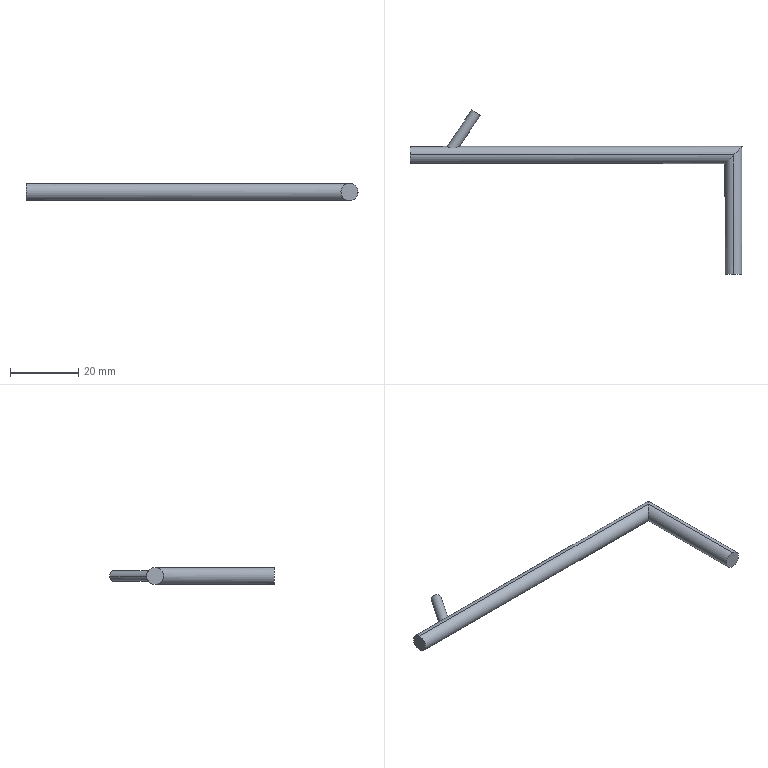Component | SolidWorks | PistonRod-1 | 1 solid | 9 faces | box 97.5 x 48.27 x 5 mm | volume 2638 mm3 | cylinder 6 | plane 3 | commonest cylinder face diameters 5 x4 3 x2
build123d program:
from build123d import *

# Parameters (mm, degrees)
SWEEP1_PROFILE_R = 2.5
SWEEP2_PROFILE_R = 1.5


with BuildPart() as part:
    # Sweep1: sweep along a path in Sketch1
    with BuildLine(Plane.XY) as sweep1_path:
        Line((35, 0), (0, 0))
        Line((0, 0), (0, 95))
    # Sweep1 profile (on start of the path) → Sweep1 (sweep)
    with BuildSketch(Plane(origin=(35, 0, 0), x_dir=(0, 0, -1), z_dir=(-1, 0, 0))):
        Circle(SWEEP1_PROFILE_R)
    sweep(path=sweep1_path.line, transition=Transition.RIGHT)

    # Sweep2: sweep along a path in Sketch2
    with BuildLine(Plane.XY) as sweep2_path:
        Line((0, 84), (-12.436, 75.612))
    # Sweep2 profile (on start of the path) → Sweep2 (sweep)
    with BuildSketch(Plane(origin=(0, 84, 0), x_dir=(0.5592, -0.829, 0), z_dir=(-0.829, -0.5592, 0))):
        Circle(SWEEP2_PROFILE_R)
    sweep(path=sweep2_path.line)


solid = part.part

# Placed as in the assembly
solid = solid.moved(Location((-25, -95, 0), (180, 0, 90)))
STEP:
#1=COLOUR_RGB('',0.7922,0.8196,0.9333);
#2=FILL_AREA_STYLE_COLOUR('',#1);
#3=FILL_AREA_STYLE('',(#2));
#4=SURFACE_STYLE_FILL_AREA(#3);
#5=SURFACE_SIDE_STYLE('',(#4));
#6=SURFACE_STYLE_USAGE(.BOTH.,#5);
#7=PRESENTATION_STYLE_ASSIGNMENT((#6));
#8=CARTESIAN_POINT('',(-4.296,-3.642,0.));
#9=VERTEX_POINT('',#8);
#10=CARTESIAN_POINT('',(-4.154,-3.642,0.));
#11=VERTEX_POINT('',#10);
#12=CARTESIAN_POINT('',(-4.296,-3.642,0.));
#13=CARTESIAN_POINT('',(-4.296,-3.642,-0.00441));
#14=CARTESIAN_POINT('',(-4.296,-3.642,-0.008751));
#15=CARTESIAN_POINT('',(-4.294,-3.643,-0.0173));
#16=CARTESIAN_POINT('',(-4.293,-3.644,-0.02152));
#17=CARTESIAN_POINT('',(-4.288,-3.647,-0.03335));
#18=CARTESIAN_POINT('',(-4.284,-3.65,-0.04043));
#19=CARTESIAN_POINT('',(-4.274,-3.655,-0.04863));
#20=CARTESIAN_POINT('',(-4.271,-3.656,-0.05101));
#21=CARTESIAN_POINT('',(-4.263,-3.658,-0.05476));
#22=CARTESIAN_POINT('',(-4.259,-3.659,-0.05621));
#23=CARTESIAN_POINT('',(-4.247,-3.661,-0.05921));
#24=CARTESIAN_POINT('',(-4.238,-3.662,-0.05945));
#25=CARTESIAN_POINT('',(-4.22,-3.66,-0.05769));
#26=CARTESIAN_POINT('',(-4.212,-3.659,-0.05569));
#27=CARTESIAN_POINT('',(-4.196,-3.655,-0.05005));
#28=CARTESIAN_POINT('',(-4.188,-3.653,-0.04641));
#29=CARTESIAN_POINT('',(-4.177,-3.65,-0.03937));
#30=CARTESIAN_POINT('',(-4.174,-3.649,-0.03679));
#31=CARTESIAN_POINT('',(-4.168,-3.647,-0.03105));
#32=CARTESIAN_POINT('',(-4.165,-3.646,-0.02785));
#33=CARTESIAN_POINT('',(-4.157,-3.643,-0.01739));
#34=CARTESIAN_POINT('',(-4.154,-3.642,-0.008908));
#35=CARTESIAN_POINT('',(-4.154,-3.642,0.));
#36=B_SPLINE_CURVE_WITH_KNOTS('',3,(#12,#13,#14,#15,#16,#17,#18,#19,#20,#21,#22,#23,#24,#25,#26,#27,#28,#29,#30,#31,#32,#33,#34,#35),.UNSPECIFIED.,.F.,.F.,(4,2,2,2,2,2,2,2,2,2,2,4),(0.005318,0.00565,0.005983,0.006647,0.00698,0.007312,0.007977,0.008641,0.009306,0.009638,0.00997,0.01064),.UNSPECIFIED.);
#37=EDGE_CURVE('',#9,#11,#36,.T.);
#38=ORIENTED_EDGE('',*,*,#37,.F.);
#39=CARTESIAN_POINT('',(-4.01,-3.218,0.));
#40=VERTEX_POINT('',#39);
#41=CARTESIAN_POINT('',(-4.34,-3.707,0.));
#42=DIRECTION('',(0.5592,0.829,-0.));
#43=VECTOR('',#42,39.37);
#44=LINE('',#41,#43);
#45=EDGE_CURVE('',#9,#40,#44,.T.);
#46=ORIENTED_EDGE('',*,*,#45,.T.);
#47=CARTESIAN_POINT('',(-3.912,-3.284,0.));
#48=VERTEX_POINT('',#47);
#49=CARTESIAN_POINT('',(-3.961,-3.251,0.));
#50=DIRECTION('',(0.5592,0.829,-0.));
#51=DIRECTION('',(0.829,-0.5592,-0.));
#52=AXIS2_PLACEMENT_3D('',#49,#50,#51);
#53=CIRCLE('',#52,0.05906);
#54=EDGE_CURVE('',#48,#40,#53,.T.);
#55=ORIENTED_EDGE('',*,*,#54,.F.);
#56=CARTESIAN_POINT('',(-4.242,-3.773,0.));
#57=DIRECTION('',(0.5592,0.829,-0.));
#58=VECTOR('',#57,39.37);
#59=LINE('',#56,#58);
#60=EDGE_CURVE('',#11,#48,#59,.T.);
#61=ORIENTED_EDGE('',*,*,#60,.F.);
#62=EDGE_LOOP('',(#38,#46,#55,#61));
#63=FACE_OUTER_BOUND('',#62,.T.);
#64=CARTESIAN_POINT('',(-4.291,-3.74,0.));
#65=DIRECTION('',(0.5592,0.829,-0.));
#66=DIRECTION('',(0.829,-0.5592,-0.));
#67=AXIS2_PLACEMENT_3D('',#64,#65,#66);
#68=CYLINDRICAL_SURFACE('',#67,0.05906);
#69=ADVANCED_FACE('',(#63),#68,.T.);
#70=CARTESIAN_POINT('',(-0.9843,-5.118,0.09843));
#71=VERTEX_POINT('',#70);
#72=CARTESIAN_POINT('',(-0.9843,-5.118,-0.09843));
#73=VERTEX_POINT('',#72);
#74=CARTESIAN_POINT('',(-0.9843,-5.118,0.));
#75=DIRECTION('',(0.,-1.,0.));
#76=DIRECTION('',(0.,0.,1.));
#77=AXIS2_PLACEMENT_3D('',#74,#75,#76);
#78=CIRCLE('',#77,0.09843);
#79=EDGE_CURVE('',#71,#73,#78,.T.);
#80=ORIENTED_EDGE('',*,*,#79,.F.);
#81=CARTESIAN_POINT('',(-0.9843,-3.74,0.09843));
#82=VERTEX_POINT('',#81);
#83=CARTESIAN_POINT('',(-0.9843,-5.118,0.09843));
#84=DIRECTION('',(0.,1.,-0.));
#85=VECTOR('',#84,39.37);
#86=LINE('',#83,#85);
#87=EDGE_CURVE('',#71,#82,#86,.T.);
#88=ORIENTED_EDGE('',*,*,#87,.T.);
#89=CARTESIAN_POINT('',(-0.9843,-3.74,-0.09843));
#90=VERTEX_POINT('',#89);
#91=CARTESIAN_POINT('',(-0.9843,-3.74,-0.09843));
#92=CARTESIAN_POINT('',(-1.181,-3.937,-0.09843));
#93=CARTESIAN_POINT('',(-1.181,-3.937,0.09843));
#94=CARTESIAN_POINT('',(-0.9843,-3.74,0.09843));
#95=(BOUNDED_CURVE()B_SPLINE_CURVE(3,(#91,#92,#93,#94),.UNSPECIFIED.,.F.,.T.)B_SPLINE_CURVE_WITH_KNOTS((4,4),(1.571,4.712),.UNSPECIFIED.)CURVE()GEOMETRIC_REPRESENTATION_ITEM()RATIONAL_B_SPLINE_CURVE((1.,0.3333,0.3333,1.))REPRESENTATION_ITEM(''));
#96=EDGE_CURVE('',#90,#82,#95,.T.);
#97=ORIENTED_EDGE('',*,*,#96,.F.);
#98=CARTESIAN_POINT('',(-0.9843,-5.118,-0.09843));
#99=DIRECTION('',(0.,1.,-0.));
#100=VECTOR('',#99,39.37);
#101=LINE('',#98,#100);
#102=EDGE_CURVE('',#73,#90,#101,.T.);
#103=ORIENTED_EDGE('',*,*,#102,.F.);
#104=EDGE_LOOP('',(#80,#88,#97,#103));
#105=FACE_OUTER_BOUND('',#104,.T.);
#106=CARTESIAN_POINT('',(-0.9843,-5.118,0.));
#107=DIRECTION('',(0.,1.,-0.));
#108=DIRECTION('',(0.,0.,-1.));
#109=AXIS2_PLACEMENT_3D('',#106,#107,#108);
#110=CYLINDRICAL_SURFACE('',#109,0.09843);
#111=ADVANCED_FACE('',(#105),#110,.T.);
#112=ORIENTED_EDGE('',*,*,#96,.T.);
#113=CARTESIAN_POINT('',(-4.724,-3.74,0.09843));
#114=VERTEX_POINT('',#113);
#115=CARTESIAN_POINT('',(-0.7638,-3.74,0.09843));
#116=DIRECTION('',(-1.,-0.,0.));
#117=VECTOR('',#116,39.37);
#118=LINE('',#115,#117);
#119=EDGE_CURVE('',#82,#114,#118,.T.);
#120=ORIENTED_EDGE('',*,*,#119,.T.);
#121=CARTESIAN_POINT('',(-4.724,-3.74,-0.09843));
#122=VERTEX_POINT('',#121);
#123=CARTESIAN_POINT('',(-4.724,-3.74,0.));
#124=DIRECTION('',(1.,0.,-0.));
#125=DIRECTION('',(0.,0.,1.));
#126=AXIS2_PLACEMENT_3D('',#123,#124,#125);
#127=CIRCLE('',#126,0.09843);
#128=EDGE_CURVE('',#114,#122,#127,.T.);
#129=ORIENTED_EDGE('',*,*,#128,.T.);
#130=CARTESIAN_POINT('',(-0.7638,-3.74,-0.09843));
#131=DIRECTION('',(-1.,-0.,0.));
#132=VECTOR('',#131,39.37);
#133=LINE('',#130,#132);
#134=EDGE_CURVE('',#90,#122,#133,.T.);
#135=ORIENTED_EDGE('',*,*,#134,.F.);
#136=EDGE_LOOP('',(#112,#120,#129,#135));
#137=FACE_OUTER_BOUND('',#136,.T.);
#138=CARTESIAN_POINT('',(-0.7638,-3.74,0.));
#139=DIRECTION('',(-1.,-0.,0.));
#140=DIRECTION('',(0.,0.,-1.));
#141=AXIS2_PLACEMENT_3D('',#138,#139,#140);
#142=CYLINDRICAL_SURFACE('',#141,0.09843);
#143=ADVANCED_FACE('',(#137),#142,.T.);
#144=ORIENTED_EDGE('',*,*,#87,.F.);
#145=CARTESIAN_POINT('',(-0.9843,-5.118,0.));
#146=DIRECTION('',(0.,-1.,0.));
#147=DIRECTION('',(0.,0.,1.));
#148=AXIS2_PLACEMENT_3D('',#145,#146,#147);
#149=CIRCLE('',#148,0.09843);
#150=EDGE_CURVE('',#73,#71,#149,.T.);
#151=ORIENTED_EDGE('',*,*,#150,.F.);
#152=ORIENTED_EDGE('',*,*,#102,.T.);
#153=CARTESIAN_POINT('',(-0.9843,-3.74,0.09843));
#154=CARTESIAN_POINT('',(-0.7874,-3.543,0.09843));
#155=CARTESIAN_POINT('',(-0.7874,-3.543,-0.09843));
#156=CARTESIAN_POINT('',(-0.9843,-3.74,-0.09843));
#157=(BOUNDED_CURVE()B_SPLINE_CURVE(3,(#153,#154,#155,#156),.UNSPECIFIED.,.F.,.T.)B_SPLINE_CURVE_WITH_KNOTS((4,4),(4.712,7.854),.UNSPECIFIED.)CURVE()GEOMETRIC_REPRESENTATION_ITEM()RATIONAL_B_SPLINE_CURVE((1.,0.3333,0.3333,1.))REPRESENTATION_ITEM(''));
#158=EDGE_CURVE('',#82,#90,#157,.T.);
#159=ORIENTED_EDGE('',*,*,#158,.F.);
#160=EDGE_LOOP('',(#144,#151,#152,#159));
#161=FACE_OUTER_BOUND('',#160,.T.);
#162=CARTESIAN_POINT('',(-0.9843,-5.118,0.));
#163=DIRECTION('',(0.,1.,-0.));
#164=DIRECTION('',(0.,0.,-1.));
#165=AXIS2_PLACEMENT_3D('',#162,#163,#164);
#166=CYLINDRICAL_SURFACE('',#165,0.09843);
#167=ADVANCED_FACE('',(#161),#166,.T.);
#168=ORIENTED_EDGE('',*,*,#119,.F.);
#169=ORIENTED_EDGE('',*,*,#158,.T.);
#170=ORIENTED_EDGE('',*,*,#134,.T.);
#171=CARTESIAN_POINT('',(-4.724,-3.74,0.));
#172=DIRECTION('',(1.,0.,-0.));
#173=DIRECTION('',(0.,0.,1.));
#174=AXIS2_PLACEMENT_3D('',#171,#172,#173);
#175=CIRCLE('',#174,0.09843);
#176=EDGE_CURVE('',#122,#114,#175,.T.);
#177=ORIENTED_EDGE('',*,*,#176,.T.);
#178=EDGE_LOOP('',(#168,#169,#170,#177));
#179=FACE_OUTER_BOUND('',#178,.T.);
#180=CARTESIAN_POINT('',(-4.154,-3.642,0.));
#181=CARTESIAN_POINT('',(-4.154,-3.642,0.00891));
#182=CARTESIAN_POINT('',(-4.157,-3.643,0.0173));
#183=CARTESIAN_POINT('',(-4.165,-3.646,0.02783));
#184=CARTESIAN_POINT('',(-4.168,-3.647,0.03101));
#185=CARTESIAN_POINT('',(-4.174,-3.649,0.03674));
#186=CARTESIAN_POINT('',(-4.177,-3.65,0.03932));
#187=CARTESIAN_POINT('',(-4.188,-3.653,0.04638));
#188=CARTESIAN_POINT('',(-4.195,-3.655,0.05002));
#189=CARTESIAN_POINT('',(-4.212,-3.659,0.05567));
#190=CARTESIAN_POINT('',(-4.22,-3.66,0.05768));
#191=CARTESIAN_POINT('',(-4.237,-3.662,0.05945));
#192=CARTESIAN_POINT('',(-4.246,-3.662,0.05922));
#193=CARTESIAN_POINT('',(-4.259,-3.659,0.05623));
#194=CARTESIAN_POINT('',(-4.263,-3.658,0.0548));
#195=CARTESIAN_POINT('',(-4.271,-3.656,0.05106));
#196=CARTESIAN_POINT('',(-4.274,-3.655,0.0487));
#197=CARTESIAN_POINT('',(-4.284,-3.65,0.04049));
#198=CARTESIAN_POINT('',(-4.288,-3.647,0.03342));
#199=CARTESIAN_POINT('',(-4.295,-3.643,0.01759));
#200=CARTESIAN_POINT('',(-4.296,-3.642,0.008821));
#201=CARTESIAN_POINT('',(-4.296,-3.642,0.));
#202=B_SPLINE_CURVE_WITH_KNOTS('',3,(#180,#181,#182,#183,#184,#185,#186,#187,#188,#189,#190,#191,#192,#193,#194,#195,#196,#197,#198,#199,#200,#201),.UNSPECIFIED.,.F.,.F.,(4,2,2,2,2,2,2,2,2,2,4),(0.,0.0006648,0.0009971,0.00133,0.001994,0.002659,0.003324,0.003656,0.003989,0.004653,0.005318),.UNSPECIFIED.);
#203=EDGE_CURVE('',#11,#9,#202,.T.);
#204=ORIENTED_EDGE('',*,*,#203,.T.);
#205=ORIENTED_EDGE('',*,*,#37,.T.);
#206=EDGE_LOOP('',(#204,#205));
#207=FACE_BOUND('',#206,.T.);
#208=CARTESIAN_POINT('',(-0.7638,-3.74,0.));
#209=DIRECTION('',(-1.,-0.,0.));
#210=DIRECTION('',(0.,0.,-1.));
#211=AXIS2_PLACEMENT_3D('',#208,#209,#210);
#212=CYLINDRICAL_SURFACE('',#211,0.09843);
#213=ADVANCED_FACE('',(#179,#207),#212,.T.);
#214=ORIENTED_EDGE('',*,*,#150,.T.);
#215=ORIENTED_EDGE('',*,*,#79,.T.);
#216=EDGE_LOOP('',(#214,#215));
#217=FACE_OUTER_BOUND('',#216,.T.);
#218=CARTESIAN_POINT('',(-0.9843,-5.118,0.));
#219=DIRECTION('',(0.,-1.,0.));
#220=DIRECTION('',(0.,0.,1.));
#221=AXIS2_PLACEMENT_3D('',#218,#219,#220);
#222=PLANE('',#221);
#223=ADVANCED_FACE('',(#217),#222,.T.);
#224=ORIENTED_EDGE('',*,*,#176,.F.);
#225=ORIENTED_EDGE('',*,*,#128,.F.);
#226=EDGE_LOOP('',(#224,#225));
#227=FACE_OUTER_BOUND('',#226,.T.);
#228=CARTESIAN_POINT('',(-4.724,-3.74,0.));
#229=DIRECTION('',(1.,0.,-0.));
#230=DIRECTION('',(0.,0.,1.));
#231=AXIS2_PLACEMENT_3D('',#228,#229,#230);
#232=PLANE('',#231);
#233=ADVANCED_FACE('',(#227),#232,.F.);
#234=ORIENTED_EDGE('',*,*,#45,.F.);
#235=ORIENTED_EDGE('',*,*,#203,.F.);
#236=ORIENTED_EDGE('',*,*,#60,.T.);
#237=CARTESIAN_POINT('',(-3.961,-3.251,0.));
#238=DIRECTION('',(0.5592,0.829,-0.));
#239=DIRECTION('',(0.829,-0.5592,-0.));
#240=AXIS2_PLACEMENT_3D('',#237,#238,#239);
#241=CIRCLE('',#240,0.05906);
#242=EDGE_CURVE('',#40,#48,#241,.T.);
#243=ORIENTED_EDGE('',*,*,#242,.F.);
#244=EDGE_LOOP('',(#234,#235,#236,#243));
#245=FACE_OUTER_BOUND('',#244,.T.);
#246=CARTESIAN_POINT('',(-4.291,-3.74,0.));
#247=DIRECTION('',(0.5592,0.829,-0.));
#248=DIRECTION('',(0.829,-0.5592,-0.));
#249=AXIS2_PLACEMENT_3D('',#246,#247,#248);
#250=CYLINDRICAL_SURFACE('',#249,0.05906);
#251=ADVANCED_FACE('',(#245),#250,.T.);
#252=ORIENTED_EDGE('',*,*,#54,.T.);
#253=ORIENTED_EDGE('',*,*,#242,.T.);
#254=EDGE_LOOP('',(#252,#253));
#255=FACE_OUTER_BOUND('',#254,.T.);
#256=CARTESIAN_POINT('',(-3.961,-3.251,0.));
#257=DIRECTION('',(0.5592,0.829,-0.));
#258=DIRECTION('',(0.829,-0.5592,-0.));
#259=AXIS2_PLACEMENT_3D('',#256,#257,#258);
#260=PLANE('',#259);
#261=ADVANCED_FACE('',(#255),#260,.T.);
#262=CLOSED_SHELL('',(#69,#111,#143,#167,#213,#223,#233,#251,#261));
#263=MANIFOLD_SOLID_BREP('',#262);
#264=STYLED_ITEM('',(#7),#263);
#265=(LENGTH_UNIT()NAMED_UNIT(*)SI_UNIT($,.METRE.));
#266=LENGTH_MEASURE_WITH_UNIT(LENGTH_MEASURE(0.0254),#265);
#267=DIMENSIONAL_EXPONENTS(1.,0.,0.,0.,0.,0.,0.);
#268=(CONVERSION_BASED_UNIT('',#266)LENGTH_UNIT()NAMED_UNIT(#267));
#269=UNCERTAINTY_MEASURE_WITH_UNIT(LENGTH_MEASURE(0.00001),#268,'','');
#270=(NAMED_UNIT(*)PLANE_ANGLE_UNIT()SI_UNIT($,.RADIAN.));
#271=(NAMED_UNIT(*)SI_UNIT($,.STERADIAN.)SOLID_ANGLE_UNIT());
#272=(GEOMETRIC_REPRESENTATION_CONTEXT(3)GLOBAL_UNCERTAINTY_ASSIGNED_CONTEXT((#269))GLOBAL_UNIT_ASSIGNED_CONTEXT((#268,#270,#271))REPRESENTATION_CONTEXT('',''));
#273=MECHANICAL_DESIGN_GEOMETRIC_PRESENTATION_REPRESENTATION('',(#264),#272);
#274=CARTESIAN_POINT('',(0.,0.,0.));
#275=DIRECTION('',(0.,0.,1.));
#276=DIRECTION('',(1.,0.,0.));
#277=AXIS2_PLACEMENT_3D('',#274,#275,#276);
#278=(LENGTH_UNIT()NAMED_UNIT(*)SI_UNIT($,.METRE.));
#279=LENGTH_MEASURE_WITH_UNIT(LENGTH_MEASURE(0.0254),#278);
#280=DIMENSIONAL_EXPONENTS(1.,0.,0.,0.,0.,0.,0.);
#281=(CONVERSION_BASED_UNIT('',#279)LENGTH_UNIT()NAMED_UNIT(#280));
#282=UNCERTAINTY_MEASURE_WITH_UNIT(LENGTH_MEASURE(0.00001),#281,'','');
#283=(NAMED_UNIT(*)PLANE_ANGLE_UNIT()SI_UNIT($,.RADIAN.));
#284=(NAMED_UNIT(*)SI_UNIT($,.STERADIAN.)SOLID_ANGLE_UNIT());
#285=(GEOMETRIC_REPRESENTATION_CONTEXT(3)GLOBAL_UNCERTAINTY_ASSIGNED_CONTEXT((#282))GLOBAL_UNIT_ASSIGNED_CONTEXT((#281,#283,#284))REPRESENTATION_CONTEXT('',''));
#286=ADVANCED_BREP_SHAPE_REPRESENTATION('',(#263,#277),#285);
#287=PRESENTATION_LAYER_ASSIGNMENT('','',(#264));